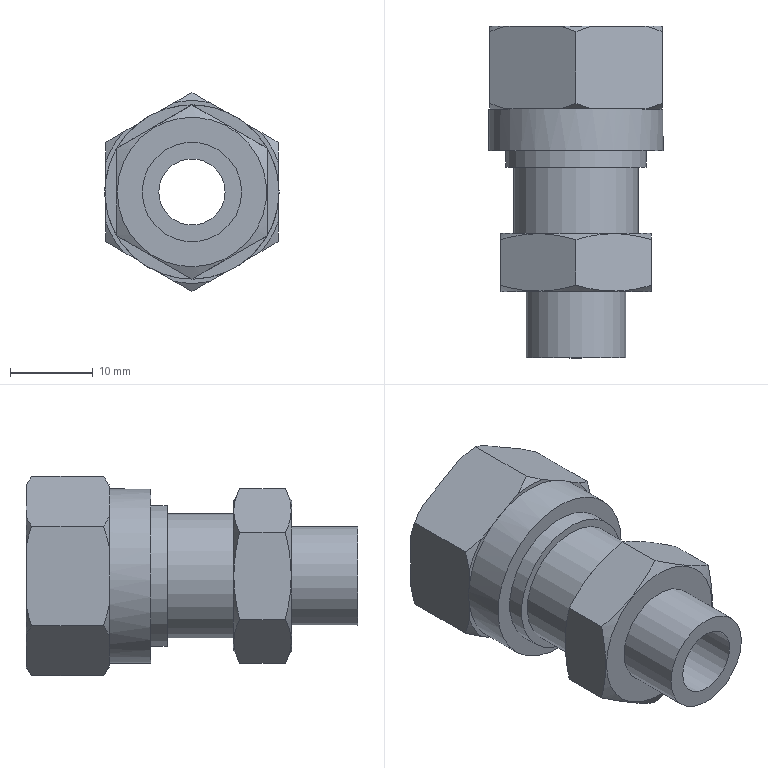Component | NX | CH3404_4-1 | 1 solid | 51 faces | volume 7647 mm3 | plane 30 | cone 15 | cylinder 6 | commonest cylinder face diameters 15 x1 17 x1 21 x1 12 x1 10 x1 8 x1